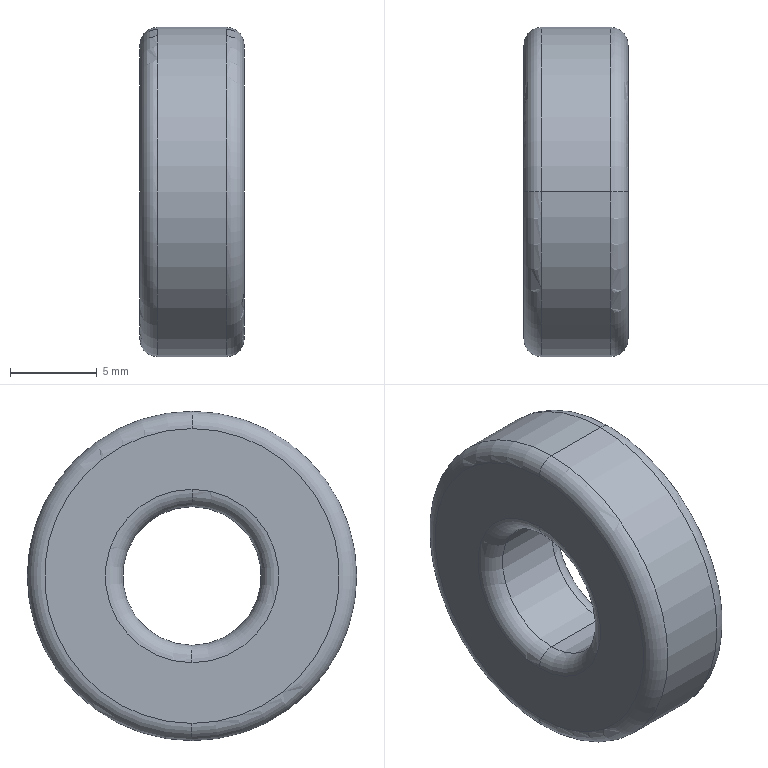Component | SolidWorks | Bearing619-8-3 | 1 solid | 14 faces | box 6 x 19 x 19 mm | volume 1363 mm3 | torus 8 | cylinder 4 | plane 2 | commonest cylinder face diameters 8 x2 19 x2
build123d program:
from build123d import *

# Parameters (mm, degrees)
SKETCH1_R           = 9.5
SKETCH1_R_2         = 4
BOSS_EXTRUDE1_DEPTH = 6
FILLET1_R           = 1


with BuildPart() as part:
    # Sketch1 → Boss-Extrude1 (new body)
    with BuildSketch(Plane.XY):
        Circle(SKETCH1_R)
        Circle(SKETCH1_R_2, mode=Mode.SUBTRACT)
    extrude(amount=BOSS_EXTRUDE1_DEPTH)

    # Fillet1
    fillet1_edges = [part.edges().sort_by_distance(p)[0] for p in [
        (-9.5, 0, 0),
        (-9.5, 0, 6),
        (-4, 0, 0),
        (-4, 0, 6),
    ]]
    fillet(fillet1_edges, radius=FILLET1_R)


solid = part.part

# Placed as in the assembly
solid = solid.moved(Location((103.726, -5.336, 80.465), (0, 90, 0)))
STEP:
#1=COLOUR_RGB('',0.7922,0.8196,0.9333);
#2=FILL_AREA_STYLE_COLOUR('',#1);
#3=FILL_AREA_STYLE('',(#2));
#4=SURFACE_STYLE_FILL_AREA(#3);
#5=SURFACE_SIDE_STYLE('',(#4));
#6=SURFACE_STYLE_USAGE(.BOTH.,#5);
#7=PRESENTATION_STYLE_ASSIGNMENT((#6));
#8=CARTESIAN_POINT('',(4.123,-0.2101,2.794));
#9=VERTEX_POINT('',#8);
#10=CARTESIAN_POINT('',(4.123,-0.2101,3.542));
#11=VERTEX_POINT('',#10);
#12=CARTESIAN_POINT('',(4.123,-0.2101,3.168));
#13=DIRECTION('',(1.,0.,-0.));
#14=DIRECTION('',(0.,0.,1.));
#15=AXIS2_PLACEMENT_3D('',#12,#13,#14);
#16=CIRCLE('',#15,0.374);
#17=EDGE_CURVE('',#9,#11,#16,.T.);
#18=ORIENTED_EDGE('',*,*,#17,.F.);
#19=CARTESIAN_POINT('',(4.084,-0.2101,2.833));
#20=VERTEX_POINT('',#19);
#21=CARTESIAN_POINT('',(4.123,-0.2101,2.833));
#22=DIRECTION('',(0.,1.,0.));
#23=DIRECTION('',(0.,0.,1.));
#24=AXIS2_PLACEMENT_3D('',#21,#22,#23);
#25=CIRCLE('',#24,0.03937);
#26=EDGE_CURVE('',#9,#20,#25,.T.);
#27=ORIENTED_EDGE('',*,*,#26,.T.);
#28=CARTESIAN_POINT('',(4.084,-0.2101,3.503));
#29=VERTEX_POINT('',#28);
#30=CARTESIAN_POINT('',(4.084,-0.2101,3.168));
#31=DIRECTION('',(-1.,0.,0.));
#32=DIRECTION('',(0.,0.,1.));
#33=AXIS2_PLACEMENT_3D('',#30,#31,#32);
#34=CIRCLE('',#33,0.3346);
#35=EDGE_CURVE('',#29,#20,#34,.T.);
#36=ORIENTED_EDGE('',*,*,#35,.F.);
#37=CARTESIAN_POINT('',(4.123,-0.2101,3.503));
#38=DIRECTION('',(0.,-1.,0.));
#39=DIRECTION('',(0.,0.,-1.));
#40=AXIS2_PLACEMENT_3D('',#37,#38,#39);
#41=CIRCLE('',#40,0.03937);
#42=EDGE_CURVE('',#11,#29,#41,.T.);
#43=ORIENTED_EDGE('',*,*,#42,.F.);
#44=EDGE_LOOP('',(#18,#27,#36,#43));
#45=FACE_OUTER_BOUND('',#44,.T.);
#46=CARTESIAN_POINT('',(4.123,-0.2101,3.168));
#47=DIRECTION('',(-1.,0.,0.));
#48=DIRECTION('',(0.,0.,1.));
#49=AXIS2_PLACEMENT_3D('',#46,#47,#48);
#50=TOROIDAL_SURFACE('',#49,0.3346,0.03937);
#51=ADVANCED_FACE('',(#45),#50,.T.);
#52=CARTESIAN_POINT('',(4.084,-0.2101,2.971));
#53=VERTEX_POINT('',#52);
#54=CARTESIAN_POINT('',(4.084,-0.2101,3.365));
#55=VERTEX_POINT('',#54);
#56=CARTESIAN_POINT('',(4.084,-0.2101,3.168));
#57=DIRECTION('',(1.,0.,-0.));
#58=DIRECTION('',(0.,0.,1.));
#59=AXIS2_PLACEMENT_3D('',#56,#57,#58);
#60=CIRCLE('',#59,0.1969);
#61=EDGE_CURVE('',#53,#55,#60,.T.);
#62=ORIENTED_EDGE('',*,*,#61,.F.);
#63=CARTESIAN_POINT('',(4.123,-0.2101,3.01));
#64=VERTEX_POINT('',#63);
#65=CARTESIAN_POINT('',(4.123,-0.2101,2.971));
#66=DIRECTION('',(0.,1.,0.));
#67=DIRECTION('',(0.,0.,1.));
#68=AXIS2_PLACEMENT_3D('',#65,#66,#67);
#69=CIRCLE('',#68,0.03937);
#70=EDGE_CURVE('',#53,#64,#69,.T.);
#71=ORIENTED_EDGE('',*,*,#70,.T.);
#72=CARTESIAN_POINT('',(4.123,-0.2101,3.325));
#73=VERTEX_POINT('',#72);
#74=CARTESIAN_POINT('',(4.123,-0.2101,3.168));
#75=DIRECTION('',(-1.,0.,0.));
#76=DIRECTION('',(0.,0.,1.));
#77=AXIS2_PLACEMENT_3D('',#74,#75,#76);
#78=CIRCLE('',#77,0.1575);
#79=EDGE_CURVE('',#73,#64,#78,.T.);
#80=ORIENTED_EDGE('',*,*,#79,.F.);
#81=CARTESIAN_POINT('',(4.123,-0.2101,3.365));
#82=DIRECTION('',(0.,-1.,0.));
#83=DIRECTION('',(0.,0.,-1.));
#84=AXIS2_PLACEMENT_3D('',#81,#82,#83);
#85=CIRCLE('',#84,0.03937);
#86=EDGE_CURVE('',#55,#73,#85,.T.);
#87=ORIENTED_EDGE('',*,*,#86,.F.);
#88=EDGE_LOOP('',(#62,#71,#80,#87));
#89=FACE_OUTER_BOUND('',#88,.T.);
#90=CARTESIAN_POINT('',(4.123,-0.2101,3.168));
#91=DIRECTION('',(-1.,0.,0.));
#92=DIRECTION('',(0.,0.,1.));
#93=AXIS2_PLACEMENT_3D('',#90,#91,#92);
#94=TOROIDAL_SURFACE('',#93,0.1969,0.03937);
#95=ADVANCED_FACE('',(#89),#94,.T.);
#96=CARTESIAN_POINT('',(4.281,-0.2101,3.01));
#97=VERTEX_POINT('',#96);
#98=CARTESIAN_POINT('',(4.281,-0.2101,3.325));
#99=VERTEX_POINT('',#98);
#100=CARTESIAN_POINT('',(4.281,-0.2101,3.168));
#101=DIRECTION('',(1.,0.,-0.));
#102=DIRECTION('',(0.,0.,1.));
#103=AXIS2_PLACEMENT_3D('',#100,#101,#102);
#104=CIRCLE('',#103,0.1575);
#105=EDGE_CURVE('',#97,#99,#104,.T.);
#106=ORIENTED_EDGE('',*,*,#105,.F.);
#107=CARTESIAN_POINT('',(4.32,-0.2101,2.971));
#108=VERTEX_POINT('',#107);
#109=CARTESIAN_POINT('',(4.281,-0.2101,2.971));
#110=DIRECTION('',(0.,1.,0.));
#111=DIRECTION('',(0.,0.,1.));
#112=AXIS2_PLACEMENT_3D('',#109,#110,#111);
#113=CIRCLE('',#112,0.03937);
#114=EDGE_CURVE('',#97,#108,#113,.T.);
#115=ORIENTED_EDGE('',*,*,#114,.T.);
#116=CARTESIAN_POINT('',(4.32,-0.2101,3.365));
#117=VERTEX_POINT('',#116);
#118=CARTESIAN_POINT('',(4.32,-0.2101,3.168));
#119=DIRECTION('',(-1.,0.,0.));
#120=DIRECTION('',(0.,0.,1.));
#121=AXIS2_PLACEMENT_3D('',#118,#119,#120);
#122=CIRCLE('',#121,0.1969);
#123=EDGE_CURVE('',#117,#108,#122,.T.);
#124=ORIENTED_EDGE('',*,*,#123,.F.);
#125=CARTESIAN_POINT('',(4.281,-0.2101,3.365));
#126=DIRECTION('',(0.,-1.,0.));
#127=DIRECTION('',(0.,0.,-1.));
#128=AXIS2_PLACEMENT_3D('',#125,#126,#127);
#129=CIRCLE('',#128,0.03937);
#130=EDGE_CURVE('',#99,#117,#129,.T.);
#131=ORIENTED_EDGE('',*,*,#130,.F.);
#132=EDGE_LOOP('',(#106,#115,#124,#131));
#133=FACE_OUTER_BOUND('',#132,.T.);
#134=CARTESIAN_POINT('',(4.281,-0.2101,3.168));
#135=DIRECTION('',(-1.,0.,0.));
#136=DIRECTION('',(0.,0.,1.));
#137=AXIS2_PLACEMENT_3D('',#134,#135,#136);
#138=TOROIDAL_SURFACE('',#137,0.1969,0.03937);
#139=ADVANCED_FACE('',(#133),#138,.T.);
#140=CARTESIAN_POINT('',(4.32,-0.2101,2.833));
#141=VERTEX_POINT('',#140);
#142=CARTESIAN_POINT('',(4.32,-0.2101,3.503));
#143=VERTEX_POINT('',#142);
#144=CARTESIAN_POINT('',(4.32,-0.2101,3.168));
#145=DIRECTION('',(1.,0.,-0.));
#146=DIRECTION('',(0.,0.,1.));
#147=AXIS2_PLACEMENT_3D('',#144,#145,#146);
#148=CIRCLE('',#147,0.3346);
#149=EDGE_CURVE('',#141,#143,#148,.T.);
#150=ORIENTED_EDGE('',*,*,#149,.F.);
#151=CARTESIAN_POINT('',(4.281,-0.2101,2.794));
#152=VERTEX_POINT('',#151);
#153=CARTESIAN_POINT('',(4.281,-0.2101,2.833));
#154=DIRECTION('',(0.,1.,0.));
#155=DIRECTION('',(0.,0.,1.));
#156=AXIS2_PLACEMENT_3D('',#153,#154,#155);
#157=CIRCLE('',#156,0.03937);
#158=EDGE_CURVE('',#141,#152,#157,.T.);
#159=ORIENTED_EDGE('',*,*,#158,.T.);
#160=CARTESIAN_POINT('',(4.281,-0.2101,3.542));
#161=VERTEX_POINT('',#160);
#162=CARTESIAN_POINT('',(4.281,-0.2101,3.168));
#163=DIRECTION('',(-1.,0.,0.));
#164=DIRECTION('',(0.,0.,1.));
#165=AXIS2_PLACEMENT_3D('',#162,#163,#164);
#166=CIRCLE('',#165,0.374);
#167=EDGE_CURVE('',#161,#152,#166,.T.);
#168=ORIENTED_EDGE('',*,*,#167,.F.);
#169=CARTESIAN_POINT('',(4.281,-0.2101,3.503));
#170=DIRECTION('',(0.,-1.,0.));
#171=DIRECTION('',(0.,0.,-1.));
#172=AXIS2_PLACEMENT_3D('',#169,#170,#171);
#173=CIRCLE('',#172,0.03937);
#174=EDGE_CURVE('',#143,#161,#173,.T.);
#175=ORIENTED_EDGE('',*,*,#174,.F.);
#176=EDGE_LOOP('',(#150,#159,#168,#175));
#177=FACE_OUTER_BOUND('',#176,.T.);
#178=CARTESIAN_POINT('',(4.281,-0.2101,3.168));
#179=DIRECTION('',(-1.,0.,0.));
#180=DIRECTION('',(0.,0.,1.));
#181=AXIS2_PLACEMENT_3D('',#178,#179,#180);
#182=TOROIDAL_SURFACE('',#181,0.3346,0.03937);
#183=ADVANCED_FACE('',(#177),#182,.T.);
#184=CARTESIAN_POINT('',(4.123,-0.2101,3.168));
#185=DIRECTION('',(-1.,0.,0.));
#186=DIRECTION('',(0.,0.,1.));
#187=AXIS2_PLACEMENT_3D('',#184,#185,#186);
#188=CIRCLE('',#187,0.1575);
#189=EDGE_CURVE('',#64,#73,#188,.T.);
#190=ORIENTED_EDGE('',*,*,#189,.T.);
#191=CARTESIAN_POINT('',(4.084,-0.2101,3.325));
#192=DIRECTION('',(1.,0.,-0.));
#193=VECTOR('',#192,39.37);
#194=LINE('',#191,#193);
#195=EDGE_CURVE('',#73,#99,#194,.T.);
#196=ORIENTED_EDGE('',*,*,#195,.T.);
#197=CARTESIAN_POINT('',(4.281,-0.2101,3.168));
#198=DIRECTION('',(1.,0.,-0.));
#199=DIRECTION('',(0.,0.,1.));
#200=AXIS2_PLACEMENT_3D('',#197,#198,#199);
#201=CIRCLE('',#200,0.1575);
#202=EDGE_CURVE('',#99,#97,#201,.T.);
#203=ORIENTED_EDGE('',*,*,#202,.T.);
#204=CARTESIAN_POINT('',(4.084,-0.2101,3.01));
#205=DIRECTION('',(1.,0.,-0.));
#206=VECTOR('',#205,39.37);
#207=LINE('',#204,#206);
#208=EDGE_CURVE('',#64,#97,#207,.T.);
#209=ORIENTED_EDGE('',*,*,#208,.F.);
#210=EDGE_LOOP('',(#190,#196,#203,#209));
#211=FACE_OUTER_BOUND('',#210,.T.);
#212=CARTESIAN_POINT('',(4.084,-0.2101,3.168));
#213=DIRECTION('',(1.,0.,-0.));
#214=DIRECTION('',(0.,0.,-1.));
#215=AXIS2_PLACEMENT_3D('',#212,#213,#214);
#216=CYLINDRICAL_SURFACE('',#215,0.1575);
#217=ADVANCED_FACE('',(#211),#216,.F.);
#218=ORIENTED_EDGE('',*,*,#17,.T.);
#219=CARTESIAN_POINT('',(4.084,-0.2101,3.542));
#220=DIRECTION('',(1.,0.,-0.));
#221=VECTOR('',#220,39.37);
#222=LINE('',#219,#221);
#223=EDGE_CURVE('',#11,#161,#222,.T.);
#224=ORIENTED_EDGE('',*,*,#223,.T.);
#225=ORIENTED_EDGE('',*,*,#167,.T.);
#226=CARTESIAN_POINT('',(4.084,-0.2101,2.794));
#227=DIRECTION('',(1.,0.,-0.));
#228=VECTOR('',#227,39.37);
#229=LINE('',#226,#228);
#230=EDGE_CURVE('',#9,#152,#229,.T.);
#231=ORIENTED_EDGE('',*,*,#230,.F.);
#232=EDGE_LOOP('',(#218,#224,#225,#231));
#233=FACE_OUTER_BOUND('',#232,.T.);
#234=CARTESIAN_POINT('',(4.084,-0.2101,3.168));
#235=DIRECTION('',(1.,0.,-0.));
#236=DIRECTION('',(0.,0.,-1.));
#237=AXIS2_PLACEMENT_3D('',#234,#235,#236);
#238=CYLINDRICAL_SURFACE('',#237,0.374);
#239=ADVANCED_FACE('',(#233),#238,.T.);
#240=CARTESIAN_POINT('',(4.084,-0.2101,3.168));
#241=DIRECTION('',(1.,0.,-0.));
#242=DIRECTION('',(0.,0.,1.));
#243=AXIS2_PLACEMENT_3D('',#240,#241,#242);
#244=CIRCLE('',#243,0.1969);
#245=EDGE_CURVE('',#55,#53,#244,.T.);
#246=ORIENTED_EDGE('',*,*,#245,.T.);
#247=ORIENTED_EDGE('',*,*,#61,.T.);
#248=EDGE_LOOP('',(#246,#247));
#249=FACE_BOUND('',#248,.T.);
#250=ORIENTED_EDGE('',*,*,#35,.T.);
#251=CARTESIAN_POINT('',(4.084,-0.2101,3.168));
#252=DIRECTION('',(-1.,0.,0.));
#253=DIRECTION('',(0.,0.,1.));
#254=AXIS2_PLACEMENT_3D('',#251,#252,#253);
#255=CIRCLE('',#254,0.3346);
#256=EDGE_CURVE('',#20,#29,#255,.T.);
#257=ORIENTED_EDGE('',*,*,#256,.T.);
#258=EDGE_LOOP('',(#250,#257));
#259=FACE_OUTER_BOUND('',#258,.T.);
#260=CARTESIAN_POINT('',(4.084,-0.2101,3.168));
#261=DIRECTION('',(-1.,0.,0.));
#262=DIRECTION('',(0.,0.,1.));
#263=AXIS2_PLACEMENT_3D('',#260,#261,#262);
#264=PLANE('',#263);
#265=ADVANCED_FACE('',(#249,#259),#264,.T.);
#266=CARTESIAN_POINT('',(4.32,-0.2101,3.168));
#267=DIRECTION('',(1.,0.,-0.));
#268=DIRECTION('',(0.,0.,1.));
#269=AXIS2_PLACEMENT_3D('',#266,#267,#268);
#270=CIRCLE('',#269,0.3346);
#271=EDGE_CURVE('',#143,#141,#270,.T.);
#272=ORIENTED_EDGE('',*,*,#271,.T.);
#273=ORIENTED_EDGE('',*,*,#149,.T.);
#274=EDGE_LOOP('',(#272,#273));
#275=FACE_OUTER_BOUND('',#274,.T.);
#276=ORIENTED_EDGE('',*,*,#123,.T.);
#277=CARTESIAN_POINT('',(4.32,-0.2101,3.168));
#278=DIRECTION('',(-1.,0.,0.));
#279=DIRECTION('',(0.,0.,1.));
#280=AXIS2_PLACEMENT_3D('',#277,#278,#279);
#281=CIRCLE('',#280,0.1969);
#282=EDGE_CURVE('',#108,#117,#281,.T.);
#283=ORIENTED_EDGE('',*,*,#282,.T.);
#284=EDGE_LOOP('',(#276,#283));
#285=FACE_BOUND('',#284,.T.);
#286=CARTESIAN_POINT('',(4.32,-0.2101,3.168));
#287=DIRECTION('',(-1.,0.,0.));
#288=DIRECTION('',(0.,0.,1.));
#289=AXIS2_PLACEMENT_3D('',#286,#287,#288);
#290=PLANE('',#289);
#291=ADVANCED_FACE('',(#275,#285),#290,.F.);
#292=ORIENTED_EDGE('',*,*,#223,.F.);
#293=CARTESIAN_POINT('',(4.123,-0.2101,3.168));
#294=DIRECTION('',(1.,0.,-0.));
#295=DIRECTION('',(0.,0.,1.));
#296=AXIS2_PLACEMENT_3D('',#293,#294,#295);
#297=CIRCLE('',#296,0.374);
#298=EDGE_CURVE('',#11,#9,#297,.T.);
#299=ORIENTED_EDGE('',*,*,#298,.T.);
#300=ORIENTED_EDGE('',*,*,#230,.T.);
#301=CARTESIAN_POINT('',(4.281,-0.2101,3.168));
#302=DIRECTION('',(-1.,0.,0.));
#303=DIRECTION('',(0.,0.,1.));
#304=AXIS2_PLACEMENT_3D('',#301,#302,#303);
#305=CIRCLE('',#304,0.374);
#306=EDGE_CURVE('',#152,#161,#305,.T.);
#307=ORIENTED_EDGE('',*,*,#306,.T.);
#308=EDGE_LOOP('',(#292,#299,#300,#307));
#309=FACE_OUTER_BOUND('',#308,.T.);
#310=CARTESIAN_POINT('',(4.084,-0.2101,3.168));
#311=DIRECTION('',(1.,0.,-0.));
#312=DIRECTION('',(0.,0.,-1.));
#313=AXIS2_PLACEMENT_3D('',#310,#311,#312);
#314=CYLINDRICAL_SURFACE('',#313,0.374);
#315=ADVANCED_FACE('',(#309),#314,.T.);
#316=ORIENTED_EDGE('',*,*,#195,.F.);
#317=ORIENTED_EDGE('',*,*,#79,.T.);
#318=ORIENTED_EDGE('',*,*,#208,.T.);
#319=ORIENTED_EDGE('',*,*,#105,.T.);
#320=EDGE_LOOP('',(#316,#317,#318,#319));
#321=FACE_OUTER_BOUND('',#320,.T.);
#322=CARTESIAN_POINT('',(4.084,-0.2101,3.168));
#323=DIRECTION('',(1.,0.,-0.));
#324=DIRECTION('',(0.,0.,-1.));
#325=AXIS2_PLACEMENT_3D('',#322,#323,#324);
#326=CYLINDRICAL_SURFACE('',#325,0.1575);
#327=ADVANCED_FACE('',(#321),#326,.F.);
#328=ORIENTED_EDGE('',*,*,#158,.F.);
#329=ORIENTED_EDGE('',*,*,#271,.F.);
#330=ORIENTED_EDGE('',*,*,#174,.T.);
#331=ORIENTED_EDGE('',*,*,#306,.F.);
#332=EDGE_LOOP('',(#328,#329,#330,#331));
#333=FACE_OUTER_BOUND('',#332,.T.);
#334=CARTESIAN_POINT('',(4.281,-0.2101,3.168));
#335=DIRECTION('',(-1.,0.,0.));
#336=DIRECTION('',(0.,0.,1.));
#337=AXIS2_PLACEMENT_3D('',#334,#335,#336);
#338=TOROIDAL_SURFACE('',#337,0.3346,0.03937);
#339=ADVANCED_FACE('',(#333),#338,.T.);
#340=ORIENTED_EDGE('',*,*,#114,.F.);
#341=ORIENTED_EDGE('',*,*,#202,.F.);
#342=ORIENTED_EDGE('',*,*,#130,.T.);
#343=ORIENTED_EDGE('',*,*,#282,.F.);
#344=EDGE_LOOP('',(#340,#341,#342,#343));
#345=FACE_OUTER_BOUND('',#344,.T.);
#346=CARTESIAN_POINT('',(4.281,-0.2101,3.168));
#347=DIRECTION('',(-1.,0.,0.));
#348=DIRECTION('',(0.,0.,1.));
#349=AXIS2_PLACEMENT_3D('',#346,#347,#348);
#350=TOROIDAL_SURFACE('',#349,0.1969,0.03937);
#351=ADVANCED_FACE('',(#345),#350,.T.);
#352=ORIENTED_EDGE('',*,*,#70,.F.);
#353=ORIENTED_EDGE('',*,*,#245,.F.);
#354=ORIENTED_EDGE('',*,*,#86,.T.);
#355=ORIENTED_EDGE('',*,*,#189,.F.);
#356=EDGE_LOOP('',(#352,#353,#354,#355));
#357=FACE_OUTER_BOUND('',#356,.T.);
#358=CARTESIAN_POINT('',(4.123,-0.2101,3.168));
#359=DIRECTION('',(-1.,0.,0.));
#360=DIRECTION('',(0.,0.,1.));
#361=AXIS2_PLACEMENT_3D('',#358,#359,#360);
#362=TOROIDAL_SURFACE('',#361,0.1969,0.03937);
#363=ADVANCED_FACE('',(#357),#362,.T.);
#364=ORIENTED_EDGE('',*,*,#26,.F.);
#365=ORIENTED_EDGE('',*,*,#298,.F.);
#366=ORIENTED_EDGE('',*,*,#42,.T.);
#367=ORIENTED_EDGE('',*,*,#256,.F.);
#368=EDGE_LOOP('',(#364,#365,#366,#367));
#369=FACE_OUTER_BOUND('',#368,.T.);
#370=CARTESIAN_POINT('',(4.123,-0.2101,3.168));
#371=DIRECTION('',(-1.,0.,0.));
#372=DIRECTION('',(0.,0.,1.));
#373=AXIS2_PLACEMENT_3D('',#370,#371,#372);
#374=TOROIDAL_SURFACE('',#373,0.3346,0.03937);
#375=ADVANCED_FACE('',(#369),#374,.T.);
#376=CLOSED_SHELL('',(#51,#95,#139,#183,#217,#239,#265,#291,#315,#327,#339,#351,#363,#375));
#377=MANIFOLD_SOLID_BREP('',#376);
#378=STYLED_ITEM('',(#7),#377);
#379=(LENGTH_UNIT()NAMED_UNIT(*)SI_UNIT($,.METRE.));
#380=LENGTH_MEASURE_WITH_UNIT(LENGTH_MEASURE(0.0254),#379);
#381=DIMENSIONAL_EXPONENTS(1.,0.,0.,0.,0.,0.,0.);
#382=(CONVERSION_BASED_UNIT('',#380)LENGTH_UNIT()NAMED_UNIT(#381));
#383=UNCERTAINTY_MEASURE_WITH_UNIT(LENGTH_MEASURE(0.00001),#382,'','');
#384=(NAMED_UNIT(*)PLANE_ANGLE_UNIT()SI_UNIT($,.RADIAN.));
#385=(NAMED_UNIT(*)SI_UNIT($,.STERADIAN.)SOLID_ANGLE_UNIT());
#386=(GEOMETRIC_REPRESENTATION_CONTEXT(3)GLOBAL_UNCERTAINTY_ASSIGNED_CONTEXT((#383))GLOBAL_UNIT_ASSIGNED_CONTEXT((#382,#384,#385))REPRESENTATION_CONTEXT('',''));
#387=MECHANICAL_DESIGN_GEOMETRIC_PRESENTATION_REPRESENTATION('',(#378),#386);
#388=PRESENTATION_LAYER_ASSIGNMENT('','',(#378));
#389=CARTESIAN_POINT('',(0.,0.,0.));
#390=DIRECTION('',(0.,0.,1.));
#391=DIRECTION('',(1.,0.,0.));
#392=AXIS2_PLACEMENT_3D('',#389,#390,#391);
#393=(LENGTH_UNIT()NAMED_UNIT(*)SI_UNIT($,.METRE.));
#394=LENGTH_MEASURE_WITH_UNIT(LENGTH_MEASURE(0.0254),#393);
#395=DIMENSIONAL_EXPONENTS(1.,0.,0.,0.,0.,0.,0.);
#396=(CONVERSION_BASED_UNIT('',#394)LENGTH_UNIT()NAMED_UNIT(#395));
#397=UNCERTAINTY_MEASURE_WITH_UNIT(LENGTH_MEASURE(0.00001),#396,'','');
#398=(NAMED_UNIT(*)PLANE_ANGLE_UNIT()SI_UNIT($,.RADIAN.));
#399=(NAMED_UNIT(*)SI_UNIT($,.STERADIAN.)SOLID_ANGLE_UNIT());
#400=(GEOMETRIC_REPRESENTATION_CONTEXT(3)GLOBAL_UNCERTAINTY_ASSIGNED_CONTEXT((#397))GLOBAL_UNIT_ASSIGNED_CONTEXT((#396,#398,#399))REPRESENTATION_CONTEXT('',''));
#401=ADVANCED_BREP_SHAPE_REPRESENTATION('',(#377,#392),#400);